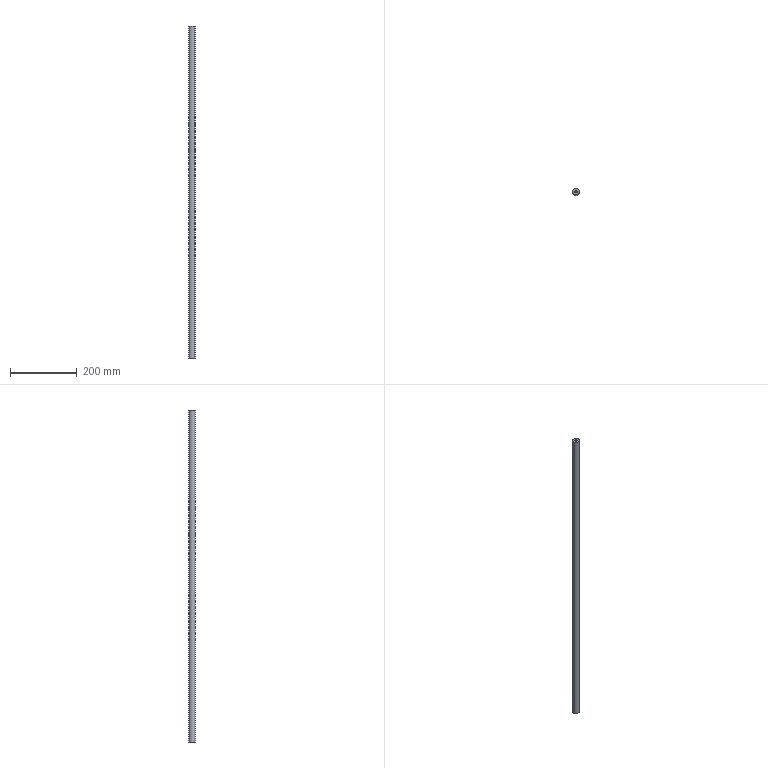Component | SolidWorks | IngotConnectingRodMandrel-1 | 1 solid | 12 faces | box 20 x 20 x 993 mm | volume 310458 mm3 | cylinder 6 | cone 4 | plane 2 | commonest cylinder face diameters 6.8 x4 20 x2
build123d program:
from build123d import *

# Parameters (mm, degrees)
BOSS_EXTRUDE1_DEPTH      = 991
BOSS_EXTRUDE1_DEPTH_BACK = 2
SKETCH1_R                = 10
M8_TAPPED_HOLE1_D        = 6.8
M8_TAPPED_HOLE1_DEPTH    = 20
M8_TAPPED_HOLE1_TIP      = 2.043
M8_TAPPED_HOLE2_D        = 6.8
M8_TAPPED_HOLE2_DEPTH    = 20
M8_TAPPED_HOLE2_TIP      = 2.043


with BuildPart() as part:
    # Sketch1 → Boss-Extrude1 (new, two sides: drawn at the far end of the back side and taken through both)
    with BuildSketch(Plane.XY.offset(-BOSS_EXTRUDE1_DEPTH_BACK)):
        with Locations((271.039, 615.177)):
            Circle(SKETCH1_R)
    extrude(amount=BOSS_EXTRUDE1_DEPTH + BOSS_EXTRUDE1_DEPTH_BACK)

    # M8 Tapped Hole1
    with Locations(Plane(origin=(271.039, 615.177, 991), x_dir=(1, 0, 0), z_dir=(0, 0, 1))):
        with Locations((0, 0)):
            Hole(M8_TAPPED_HOLE1_D / 2, depth=M8_TAPPED_HOLE1_DEPTH)
            with Locations((0, 0, -(M8_TAPPED_HOLE1_DEPTH + M8_TAPPED_HOLE1_TIP / 2))):  # 118° drill point
                Cone(0, M8_TAPPED_HOLE1_D / 2, M8_TAPPED_HOLE1_TIP, mode=Mode.SUBTRACT)

    # M8 Tapped Hole2
    with Locations(Plane(origin=(271.039, 615.177, -2), x_dir=(-1, 0, 0), z_dir=(0, 0, -1))):
        with Locations((0, 0)):
            Hole(M8_TAPPED_HOLE2_D / 2, depth=M8_TAPPED_HOLE2_DEPTH)
            with Locations((0, 0, -(M8_TAPPED_HOLE2_DEPTH + M8_TAPPED_HOLE2_TIP / 2))):  # 118° drill point
                Cone(0, M8_TAPPED_HOLE2_D / 2, M8_TAPPED_HOLE2_TIP, mode=Mode.SUBTRACT)


solid = part.part

# Placed as in the assembly
solid = solid.moved(Location((0, 0, 0.5), (0, 0, 0)))
STEP:
#1=CARTESIAN_POINT('',(10.759,24.119,0.7283));
#2=VERTEX_POINT('',#1);
#3=CARTESIAN_POINT('',(10.583,24.32,0.7283));
#4=VERTEX_POINT('',#3);
#5=CARTESIAN_POINT('',(10.671,24.22,0.7283));
#6=DIRECTION('',(0.,0.,-1.));
#7=DIRECTION('',(-0.659,0.7522,0.));
#8=AXIS2_PLACEMENT_3D('',#5,#6,#7);
#9=CIRCLE('',#8,0.1339);
#10=EDGE_CURVE('',#2,#4,#9,.T.);
#11=ORIENTED_EDGE('',*,*,#10,.F.);
#12=CARTESIAN_POINT('',(10.759,24.119,-0.05906));
#13=VERTEX_POINT('',#12);
#14=CARTESIAN_POINT('',(10.759,24.119,-0.05906));
#15=DIRECTION('',(0.,0.,-1.));
#16=VECTOR('',#15,39.37);
#17=LINE('',#14,#16);
#18=EDGE_CURVE('',#2,#13,#17,.T.);
#19=ORIENTED_EDGE('',*,*,#18,.T.);
#20=CARTESIAN_POINT('',(10.583,24.32,-0.05906));
#21=VERTEX_POINT('',#20);
#22=CARTESIAN_POINT('',(10.671,24.22,-0.05906));
#23=DIRECTION('',(0.,0.,-1.));
#24=DIRECTION('',(-0.659,0.7522,0.));
#25=AXIS2_PLACEMENT_3D('',#22,#23,#24);
#26=CIRCLE('',#25,0.1339);
#27=EDGE_CURVE('',#13,#21,#26,.T.);
#28=ORIENTED_EDGE('',*,*,#27,.T.);
#29=CARTESIAN_POINT('',(10.583,24.32,-0.05906));
#30=DIRECTION('',(0.,0.,-1.));
#31=VECTOR('',#30,39.37);
#32=LINE('',#29,#31);
#33=EDGE_CURVE('',#4,#21,#32,.T.);
#34=ORIENTED_EDGE('',*,*,#33,.F.);
#35=EDGE_LOOP('',(#11,#19,#28,#34));
#36=FACE_OUTER_BOUND('',#35,.T.);
#37=CARTESIAN_POINT('',(10.671,24.22,-0.05906));
#38=DIRECTION('',(0.,0.,-1.));
#39=DIRECTION('',(-0.659,0.7522,0.));
#40=AXIS2_PLACEMENT_3D('',#37,#38,#39);
#41=CYLINDRICAL_SURFACE('',#40,0.1339);
#42=ADVANCED_FACE('',(#36),#41,.F.);
#43=CARTESIAN_POINT('',(10.671,24.22,0.8088));
#44=VERTEX_POINT('',#43);
#45=CARTESIAN_POINT('',(10.583,24.32,0.7283));
#46=DIRECTION('',(-0.5649,0.6447,-0.515));
#47=VECTOR('',#46,39.37);
#48=LINE('',#45,#47);
#49=EDGE_CURVE('',#44,#4,#48,.T.);
#50=ORIENTED_EDGE('',*,*,#49,.F.);
#51=CARTESIAN_POINT('',(10.759,24.119,0.7283));
#52=DIRECTION('',(0.5649,-0.6447,-0.515));
#53=VECTOR('',#52,39.37);
#54=LINE('',#51,#53);
#55=EDGE_CURVE('',#44,#2,#54,.T.);
#56=ORIENTED_EDGE('',*,*,#55,.T.);
#57=ORIENTED_EDGE('',*,*,#10,.T.);
#58=EDGE_LOOP('',(#50,#56,#57));
#59=FACE_OUTER_BOUND('',#58,.T.);
#60=CARTESIAN_POINT('',(10.671,24.22,0.7283));
#61=DIRECTION('',(0.,0.,-1.));
#62=DIRECTION('',(-0.659,0.7522,0.));
#63=AXIS2_PLACEMENT_3D('',#60,#61,#62);
#64=CONICAL_SURFACE('',#63,0.1339,1.03);
#65=ADVANCED_FACE('',(#59),#64,.F.);
#66=CARTESIAN_POINT('',(10.583,24.32,38.248));
#67=VERTEX_POINT('',#66);
#68=CARTESIAN_POINT('',(10.759,24.119,38.248));
#69=VERTEX_POINT('',#68);
#70=CARTESIAN_POINT('',(10.671,24.22,38.248));
#71=DIRECTION('',(0.,0.,1.));
#72=DIRECTION('',(0.659,-0.7522,0.));
#73=AXIS2_PLACEMENT_3D('',#70,#71,#72);
#74=CIRCLE('',#73,0.1339);
#75=EDGE_CURVE('',#67,#69,#74,.T.);
#76=ORIENTED_EDGE('',*,*,#75,.F.);
#77=CARTESIAN_POINT('',(10.583,24.32,39.035));
#78=VERTEX_POINT('',#77);
#79=CARTESIAN_POINT('',(10.583,24.32,39.035));
#80=DIRECTION('',(0.,0.,1.));
#81=VECTOR('',#80,39.37);
#82=LINE('',#79,#81);
#83=EDGE_CURVE('',#67,#78,#82,.T.);
#84=ORIENTED_EDGE('',*,*,#83,.T.);
#85=CARTESIAN_POINT('',(10.759,24.119,39.035));
#86=VERTEX_POINT('',#85);
#87=CARTESIAN_POINT('',(10.671,24.22,39.035));
#88=DIRECTION('',(0.,0.,1.));
#89=DIRECTION('',(0.659,-0.7522,0.));
#90=AXIS2_PLACEMENT_3D('',#87,#88,#89);
#91=CIRCLE('',#90,0.1339);
#92=EDGE_CURVE('',#78,#86,#91,.T.);
#93=ORIENTED_EDGE('',*,*,#92,.T.);
#94=CARTESIAN_POINT('',(10.759,24.119,39.035));
#95=DIRECTION('',(0.,0.,1.));
#96=VECTOR('',#95,39.37);
#97=LINE('',#94,#96);
#98=EDGE_CURVE('',#69,#86,#97,.T.);
#99=ORIENTED_EDGE('',*,*,#98,.F.);
#100=EDGE_LOOP('',(#76,#84,#93,#99));
#101=FACE_OUTER_BOUND('',#100,.T.);
#102=CARTESIAN_POINT('',(10.671,24.22,39.035));
#103=DIRECTION('',(0.,0.,1.));
#104=DIRECTION('',(0.659,-0.7522,0.));
#105=AXIS2_PLACEMENT_3D('',#102,#103,#104);
#106=CYLINDRICAL_SURFACE('',#105,0.1339);
#107=ADVANCED_FACE('',(#101),#106,.F.);
#108=CARTESIAN_POINT('',(10.671,24.22,38.168));
#109=VERTEX_POINT('',#108);
#110=CARTESIAN_POINT('',(10.759,24.119,38.248));
#111=DIRECTION('',(0.5649,-0.6447,0.515));
#112=VECTOR('',#111,39.37);
#113=LINE('',#110,#112);
#114=EDGE_CURVE('',#109,#69,#113,.T.);
#115=ORIENTED_EDGE('',*,*,#114,.F.);
#116=CARTESIAN_POINT('',(10.583,24.32,38.248));
#117=DIRECTION('',(-0.5649,0.6447,0.515));
#118=VECTOR('',#117,39.37);
#119=LINE('',#116,#118);
#120=EDGE_CURVE('',#109,#67,#119,.T.);
#121=ORIENTED_EDGE('',*,*,#120,.T.);
#122=ORIENTED_EDGE('',*,*,#75,.T.);
#123=EDGE_LOOP('',(#115,#121,#122));
#124=FACE_OUTER_BOUND('',#123,.T.);
#125=CARTESIAN_POINT('',(10.671,24.22,38.248));
#126=DIRECTION('',(0.,0.,1.));
#127=DIRECTION('',(0.659,-0.7522,0.));
#128=AXIS2_PLACEMENT_3D('',#125,#126,#127);
#129=CONICAL_SURFACE('',#128,0.1339,1.03);
#130=ADVANCED_FACE('',(#124),#129,.F.);
#131=CARTESIAN_POINT('',(10.93,23.923,-0.05906));
#132=VERTEX_POINT('',#131);
#133=CARTESIAN_POINT('',(10.411,24.516,-0.05906));
#134=VERTEX_POINT('',#133);
#135=CARTESIAN_POINT('',(10.671,24.22,-0.05906));
#136=DIRECTION('',(0.,0.,1.));
#137=DIRECTION('',(0.659,-0.7522,0.));
#138=AXIS2_PLACEMENT_3D('',#135,#136,#137);
#139=CIRCLE('',#138,0.3937);
#140=EDGE_CURVE('',#132,#134,#139,.T.);
#141=ORIENTED_EDGE('',*,*,#140,.T.);
#142=CARTESIAN_POINT('',(10.411,24.516,39.035));
#143=VERTEX_POINT('',#142);
#144=CARTESIAN_POINT('',(10.411,24.516,-0.05906));
#145=DIRECTION('',(0.,0.,1.));
#146=VECTOR('',#145,39.37);
#147=LINE('',#144,#146);
#148=EDGE_CURVE('',#134,#143,#147,.T.);
#149=ORIENTED_EDGE('',*,*,#148,.T.);
#150=CARTESIAN_POINT('',(10.93,23.923,39.035));
#151=VERTEX_POINT('',#150);
#152=CARTESIAN_POINT('',(10.671,24.22,39.035));
#153=DIRECTION('',(0.,0.,1.));
#154=DIRECTION('',(0.659,-0.7522,0.));
#155=AXIS2_PLACEMENT_3D('',#152,#153,#154);
#156=CIRCLE('',#155,0.3937);
#157=EDGE_CURVE('',#151,#143,#156,.T.);
#158=ORIENTED_EDGE('',*,*,#157,.F.);
#159=CARTESIAN_POINT('',(10.93,23.923,-0.05906));
#160=DIRECTION('',(0.,0.,1.));
#161=VECTOR('',#160,39.37);
#162=LINE('',#159,#161);
#163=EDGE_CURVE('',#132,#151,#162,.T.);
#164=ORIENTED_EDGE('',*,*,#163,.F.);
#165=EDGE_LOOP('',(#141,#149,#158,#164));
#166=FACE_OUTER_BOUND('',#165,.T.);
#167=CARTESIAN_POINT('',(10.671,24.22,-0.05906));
#168=DIRECTION('',(0.,0.,1.));
#169=DIRECTION('',(0.659,-0.7522,0.));
#170=AXIS2_PLACEMENT_3D('',#167,#168,#169);
#171=CYLINDRICAL_SURFACE('',#170,0.3937);
#172=ADVANCED_FACE('',(#166),#171,.T.);
#173=ORIENTED_EDGE('',*,*,#148,.F.);
#174=CARTESIAN_POINT('',(10.671,24.22,-0.05906));
#175=DIRECTION('',(0.,0.,1.));
#176=DIRECTION('',(0.659,-0.7522,0.));
#177=AXIS2_PLACEMENT_3D('',#174,#175,#176);
#178=CIRCLE('',#177,0.3937);
#179=EDGE_CURVE('',#134,#132,#178,.T.);
#180=ORIENTED_EDGE('',*,*,#179,.T.);
#181=ORIENTED_EDGE('',*,*,#163,.T.);
#182=CARTESIAN_POINT('',(10.671,24.22,39.035));
#183=DIRECTION('',(0.,0.,1.));
#184=DIRECTION('',(0.659,-0.7522,0.));
#185=AXIS2_PLACEMENT_3D('',#182,#183,#184);
#186=CIRCLE('',#185,0.3937);
#187=EDGE_CURVE('',#143,#151,#186,.T.);
#188=ORIENTED_EDGE('',*,*,#187,.F.);
#189=EDGE_LOOP('',(#173,#180,#181,#188));
#190=FACE_OUTER_BOUND('',#189,.T.);
#191=CARTESIAN_POINT('',(10.671,24.22,-0.05906));
#192=DIRECTION('',(0.,0.,1.));
#193=DIRECTION('',(0.659,-0.7522,0.));
#194=AXIS2_PLACEMENT_3D('',#191,#192,#193);
#195=CYLINDRICAL_SURFACE('',#194,0.3937);
#196=ADVANCED_FACE('',(#190),#195,.T.);
#197=CARTESIAN_POINT('',(10.671,24.22,-0.05906));
#198=DIRECTION('',(0.,0.,-1.));
#199=DIRECTION('',(-0.659,0.7522,0.));
#200=AXIS2_PLACEMENT_3D('',#197,#198,#199);
#201=CIRCLE('',#200,0.1339);
#202=EDGE_CURVE('',#21,#13,#201,.T.);
#203=ORIENTED_EDGE('',*,*,#202,.F.);
#204=ORIENTED_EDGE('',*,*,#27,.F.);
#205=EDGE_LOOP('',(#203,#204));
#206=FACE_BOUND('',#205,.T.);
#207=ORIENTED_EDGE('',*,*,#140,.F.);
#208=ORIENTED_EDGE('',*,*,#179,.F.);
#209=EDGE_LOOP('',(#207,#208));
#210=FACE_OUTER_BOUND('',#209,.T.);
#211=CARTESIAN_POINT('',(10.671,24.22,-0.05906));
#212=DIRECTION('',(0.,0.,1.));
#213=DIRECTION('',(0.659,-0.7522,0.));
#214=AXIS2_PLACEMENT_3D('',#211,#212,#213);
#215=PLANE('',#214);
#216=ADVANCED_FACE('',(#206,#210),#215,.F.);
#217=CARTESIAN_POINT('',(10.671,24.22,39.035));
#218=DIRECTION('',(0.,0.,1.));
#219=DIRECTION('',(0.659,-0.7522,0.));
#220=AXIS2_PLACEMENT_3D('',#217,#218,#219);
#221=CIRCLE('',#220,0.1339);
#222=EDGE_CURVE('',#86,#78,#221,.T.);
#223=ORIENTED_EDGE('',*,*,#222,.F.);
#224=ORIENTED_EDGE('',*,*,#92,.F.);
#225=EDGE_LOOP('',(#223,#224));
#226=FACE_BOUND('',#225,.T.);
#227=ORIENTED_EDGE('',*,*,#157,.T.);
#228=ORIENTED_EDGE('',*,*,#187,.T.);
#229=EDGE_LOOP('',(#227,#228));
#230=FACE_OUTER_BOUND('',#229,.T.);
#231=CARTESIAN_POINT('',(10.671,24.22,39.035));
#232=DIRECTION('',(0.,0.,1.));
#233=DIRECTION('',(0.659,-0.7522,0.));
#234=AXIS2_PLACEMENT_3D('',#231,#232,#233);
#235=PLANE('',#234);
#236=ADVANCED_FACE('',(#226,#230),#235,.T.);
#237=ORIENTED_EDGE('',*,*,#120,.F.);
#238=ORIENTED_EDGE('',*,*,#114,.T.);
#239=CARTESIAN_POINT('',(10.671,24.22,38.248));
#240=DIRECTION('',(0.,0.,1.));
#241=DIRECTION('',(0.659,-0.7522,0.));
#242=AXIS2_PLACEMENT_3D('',#239,#240,#241);
#243=CIRCLE('',#242,0.1339);
#244=EDGE_CURVE('',#69,#67,#243,.T.);
#245=ORIENTED_EDGE('',*,*,#244,.T.);
#246=EDGE_LOOP('',(#237,#238,#245));
#247=FACE_OUTER_BOUND('',#246,.T.);
#248=CARTESIAN_POINT('',(10.671,24.22,38.248));
#249=DIRECTION('',(0.,0.,1.));
#250=DIRECTION('',(0.659,-0.7522,0.));
#251=AXIS2_PLACEMENT_3D('',#248,#249,#250);
#252=CONICAL_SURFACE('',#251,0.1339,1.03);
#253=ADVANCED_FACE('',(#247),#252,.F.);
#254=ORIENTED_EDGE('',*,*,#83,.F.);
#255=ORIENTED_EDGE('',*,*,#244,.F.);
#256=ORIENTED_EDGE('',*,*,#98,.T.);
#257=ORIENTED_EDGE('',*,*,#222,.T.);
#258=EDGE_LOOP('',(#254,#255,#256,#257));
#259=FACE_OUTER_BOUND('',#258,.T.);
#260=CARTESIAN_POINT('',(10.671,24.22,39.035));
#261=DIRECTION('',(0.,0.,1.));
#262=DIRECTION('',(0.659,-0.7522,0.));
#263=AXIS2_PLACEMENT_3D('',#260,#261,#262);
#264=CYLINDRICAL_SURFACE('',#263,0.1339);
#265=ADVANCED_FACE('',(#259),#264,.F.);
#266=ORIENTED_EDGE('',*,*,#55,.F.);
#267=ORIENTED_EDGE('',*,*,#49,.T.);
#268=CARTESIAN_POINT('',(10.671,24.22,0.7283));
#269=DIRECTION('',(0.,0.,-1.));
#270=DIRECTION('',(-0.659,0.7522,0.));
#271=AXIS2_PLACEMENT_3D('',#268,#269,#270);
#272=CIRCLE('',#271,0.1339);
#273=EDGE_CURVE('',#4,#2,#272,.T.);
#274=ORIENTED_EDGE('',*,*,#273,.T.);
#275=EDGE_LOOP('',(#266,#267,#274));
#276=FACE_OUTER_BOUND('',#275,.T.);
#277=CARTESIAN_POINT('',(10.671,24.22,0.7283));
#278=DIRECTION('',(0.,0.,-1.));
#279=DIRECTION('',(-0.659,0.7522,0.));
#280=AXIS2_PLACEMENT_3D('',#277,#278,#279);
#281=CONICAL_SURFACE('',#280,0.1339,1.03);
#282=ADVANCED_FACE('',(#276),#281,.F.);
#283=ORIENTED_EDGE('',*,*,#18,.F.);
#284=ORIENTED_EDGE('',*,*,#273,.F.);
#285=ORIENTED_EDGE('',*,*,#33,.T.);
#286=ORIENTED_EDGE('',*,*,#202,.T.);
#287=EDGE_LOOP('',(#283,#284,#285,#286));
#288=FACE_OUTER_BOUND('',#287,.T.);
#289=CARTESIAN_POINT('',(10.671,24.22,-0.05906));
#290=DIRECTION('',(0.,0.,-1.));
#291=DIRECTION('',(-0.659,0.7522,0.));
#292=AXIS2_PLACEMENT_3D('',#289,#290,#291);
#293=CYLINDRICAL_SURFACE('',#292,0.1339);
#294=ADVANCED_FACE('',(#288),#293,.F.);
#295=CLOSED_SHELL('',(#42,#65,#107,#130,#172,#196,#216,#236,#253,#265,#282,#294));
#296=MANIFOLD_SOLID_BREP('',#295);
#297=CARTESIAN_POINT('',(0.,0.,0.));
#298=DIRECTION('',(0.,0.,1.));
#299=DIRECTION('',(1.,0.,0.));
#300=AXIS2_PLACEMENT_3D('',#297,#298,#299);
#301=(LENGTH_UNIT()NAMED_UNIT(*)SI_UNIT($,.METRE.));
#302=LENGTH_MEASURE_WITH_UNIT(LENGTH_MEASURE(0.0254),#301);
#303=DIMENSIONAL_EXPONENTS(1.,0.,0.,0.,0.,0.,0.);
#304=(CONVERSION_BASED_UNIT('',#302)LENGTH_UNIT()NAMED_UNIT(#303));
#305=UNCERTAINTY_MEASURE_WITH_UNIT(LENGTH_MEASURE(0.00001),#304,'','');
#306=(NAMED_UNIT(*)PLANE_ANGLE_UNIT()SI_UNIT($,.RADIAN.));
#307=(NAMED_UNIT(*)SI_UNIT($,.STERADIAN.)SOLID_ANGLE_UNIT());
#308=(GEOMETRIC_REPRESENTATION_CONTEXT(3)GLOBAL_UNCERTAINTY_ASSIGNED_CONTEXT((#305))GLOBAL_UNIT_ASSIGNED_CONTEXT((#304,#306,#307))REPRESENTATION_CONTEXT('',''));
#309=ADVANCED_BREP_SHAPE_REPRESENTATION('',(#296,#300),#308);
#310=COLOUR_RGB('',0.7922,0.8196,0.9333);
#311=FILL_AREA_STYLE_COLOUR('',#310);
#312=FILL_AREA_STYLE('',(#311));
#313=SURFACE_STYLE_FILL_AREA(#312);
#314=SURFACE_SIDE_STYLE('',(#313));
#315=SURFACE_STYLE_USAGE(.BOTH.,#314);
#316=PRESENTATION_STYLE_ASSIGNMENT((#315));
#317=STYLED_ITEM('',(#316),#296);
#318=PRESENTATION_LAYER_ASSIGNMENT('','',(#317));
#319=(LENGTH_UNIT()NAMED_UNIT(*)SI_UNIT($,.METRE.));
#320=LENGTH_MEASURE_WITH_UNIT(LENGTH_MEASURE(0.0254),#319);
#321=DIMENSIONAL_EXPONENTS(1.,0.,0.,0.,0.,0.,0.);
#322=(CONVERSION_BASED_UNIT('',#320)LENGTH_UNIT()NAMED_UNIT(#321));
#323=UNCERTAINTY_MEASURE_WITH_UNIT(LENGTH_MEASURE(0.00001),#322,'','');
#324=(NAMED_UNIT(*)PLANE_ANGLE_UNIT()SI_UNIT($,.RADIAN.));
#325=(NAMED_UNIT(*)SI_UNIT($,.STERADIAN.)SOLID_ANGLE_UNIT());
#326=(GEOMETRIC_REPRESENTATION_CONTEXT(3)GLOBAL_UNCERTAINTY_ASSIGNED_CONTEXT((#323))GLOBAL_UNIT_ASSIGNED_CONTEXT((#322,#324,#325))REPRESENTATION_CONTEXT('',''));
#327=MECHANICAL_DESIGN_GEOMETRIC_PRESENTATION_REPRESENTATION('',(#317),#326);